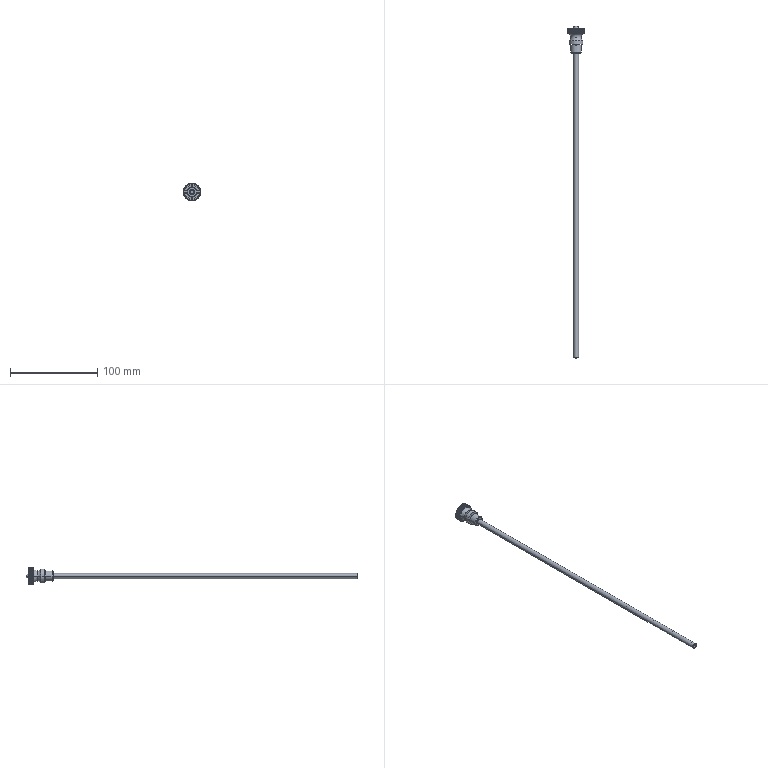Component | SolidWorks | OilGauge-1 | 1 solid | 269 faces | volume 13343 mm3 | plane 187 | cylinder 70 | cone 6 | torus 4 | sphere 2 | commonest cylinder face diameters 20 x60 4 x2 6 x2 16 x2 9 x2 12 x2